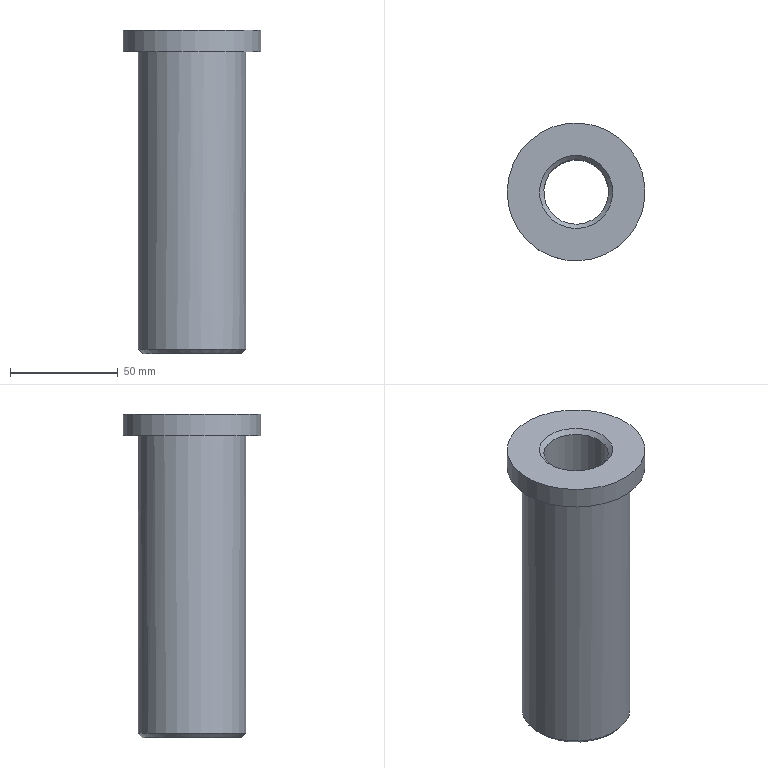Component | NX | PRESSURE_BUSHING | 1 solid | 9 faces | box 64 x 64 x 150 mm | volume 200331 mm3 | plane 3 | cylinder 3 | cone 3 | commonest cylinder face diameters 30 x1 64 x1 50 x1
STEP:
#1=CARTESIAN_POINT('',(0.,0.,0.));
#2=DIRECTION('',(0.,0.,1.));
#3=DIRECTION('',(1.,0.,0.));
#4=AXIS2_PLACEMENT_3D('',#1,#2,#3);
#5=CARTESIAN_POINT('',(-209.297,6.512,90.));
#6=VERTEX_POINT('',#5);
#7=CARTESIAN_POINT('',(-225.,0.,90.));
#8=DIRECTION('',(0.,0.,1.));
#9=DIRECTION('',(0.9237,0.383,0.));
#10=AXIS2_PLACEMENT_3D('',#7,#8,#9);
#11=CIRCLE('',#10,17.);
#12=CARTESIAN_POINT('',(-234.576,23.093,90.));
#13=DIRECTION('',(0.,0.,1.));
#14=DIRECTION('',(0.9237,0.383,0.));
#15=AXIS2_PLACEMENT_3D('',#12,#13,#14);
#16=PLANE('',#15);
#17=CARTESIAN_POINT('',(0.,-25.));
#18=DIRECTION('',(1.,0.));
#19=AXIS2_PLACEMENT_2D('',#17,#18);
#20=CIRCLE('',#19,17.);
#21=(GEOMETRIC_REPRESENTATION_CONTEXT(2)PARAMETRIC_REPRESENTATION_CONTEXT()REPRESENTATION_CONTEXT('',''));
#22=DEFINITIONAL_REPRESENTATION('',(#20),#21);
#23=PCURVE('',#16,#22);
#24=CARTESIAN_POINT('',(-225.,0.,92.));
#25=DIRECTION('',(0.,0.,-1.));
#26=DIRECTION('',(-0.9237,-0.383,0.));
#27=AXIS2_PLACEMENT_3D('',#24,#25,#26);
#28=CONICAL_SURFACE('',#27,15.,0.7854);
#29=CARTESIAN_POINT('',(9.425,2.));
#30=DIRECTION('',(-1.,0.));
#31=VECTOR('',#30,1.);
#32=LINE('',#29,#31);
#33=(GEOMETRIC_REPRESENTATION_CONTEXT(2)PARAMETRIC_REPRESENTATION_CONTEXT()REPRESENTATION_CONTEXT('',''));
#34=DEFINITIONAL_REPRESENTATION('',(#32),#33);
#35=PCURVE('',#28,#34);
#36=SURFACE_CURVE('',#11,(#23,#35),.PCURVE_S1.);
#37=EDGE_CURVE('',#6,#6,#36,.T.);
#38=ORIENTED_EDGE('',*,*,#37,.T.);
#39=EDGE_LOOP('',(#38));
#40=FACE_BOUND('',#39,.T.);
#41=CARTESIAN_POINT('',(-203.754,8.81,90.));
#42=VERTEX_POINT('',#41);
#43=CARTESIAN_POINT('',(-225.,0.,90.));
#44=DIRECTION('',(0.,0.,-1.));
#45=DIRECTION('',(0.9237,0.383,0.));
#46=AXIS2_PLACEMENT_3D('',#43,#44,#45);
#47=CIRCLE('',#46,23.);
#48=CARTESIAN_POINT('',(23.,-25.));
#49=CARTESIAN_POINT('',(23.,-64.837));
#50=CARTESIAN_POINT('',(-11.5,-44.919));
#51=CARTESIAN_POINT('',(-46.,-25.));
#52=CARTESIAN_POINT('',(-11.5,-5.081));
#53=CARTESIAN_POINT('',(23.,14.837));
#54=CARTESIAN_POINT('',(23.,-25.));
#55=(BOUNDED_CURVE()B_SPLINE_CURVE(2,(#48,#49,#50,#51,#52,#53,#54),.UNSPECIFIED.,.T.,.F.)B_SPLINE_CURVE_WITH_KNOTS((1,2,2,2,2,1),(-2.094,0.,2.094,4.189,6.283,8.378),.UNSPECIFIED.)CURVE()GEOMETRIC_REPRESENTATION_ITEM()RATIONAL_B_SPLINE_CURVE((1.,0.5,1.,0.5,1.,0.5,1.))REPRESENTATION_ITEM(''));
#56=(GEOMETRIC_REPRESENTATION_CONTEXT(2)PARAMETRIC_REPRESENTATION_CONTEXT()REPRESENTATION_CONTEXT('',''));
#57=DEFINITIONAL_REPRESENTATION('',(#55),#56);
#58=PCURVE('',#16,#57);
#59=CARTESIAN_POINT('',(-225.,0.,90.));
#60=DIRECTION('',(0.,0.,1.));
#61=DIRECTION('',(0.9237,0.383,0.));
#62=AXIS2_PLACEMENT_3D('',#59,#60,#61);
#63=CONICAL_SURFACE('',#62,23.,0.7854);
#64=CARTESIAN_POINT('',(6.283,-0.));
#65=DIRECTION('',(-1.,0.));
#66=VECTOR('',#65,1.);
#67=LINE('',#64,#66);
#68=(GEOMETRIC_REPRESENTATION_CONTEXT(2)PARAMETRIC_REPRESENTATION_CONTEXT()REPRESENTATION_CONTEXT('',''));
#69=DEFINITIONAL_REPRESENTATION('',(#67),#68);
#70=PCURVE('',#63,#69);
#71=SURFACE_CURVE('',#47,(#58,#70),.PCURVE_S1.);
#72=EDGE_CURVE('',#42,#42,#71,.T.);
#73=ORIENTED_EDGE('',*,*,#72,.T.);
#74=EDGE_LOOP('',(#73));
#75=FACE_BOUND('',#74,.T.);
#76=ADVANCED_FACE('',(#40,#75),#16,.F.);
#77=CARTESIAN_POINT('',(-238.856,-5.746,92.));
#78=VERTEX_POINT('',#77);
#79=CARTESIAN_POINT('',(-211.144,5.746,92.));
#80=VERTEX_POINT('',#79);
#81=CARTESIAN_POINT('',(-225.,0.,92.));
#82=DIRECTION('',(0.,0.,-1.));
#83=DIRECTION('',(0.9237,0.383,0.));
#84=AXIS2_PLACEMENT_3D('',#81,#82,#83);
#85=CIRCLE('',#84,15.);
#86=CARTESIAN_POINT('',(-225.,0.,230.));
#87=DIRECTION('',(0.,0.,-1.));
#88=DIRECTION('',(-0.9237,-0.383,0.));
#89=AXIS2_PLACEMENT_3D('',#86,#87,#88);
#90=CYLINDRICAL_SURFACE('',#89,15.);
#91=CARTESIAN_POINT('',(-3.142,138.));
#92=DIRECTION('',(1.,0.));
#93=VECTOR('',#92,1.);
#94=LINE('',#91,#93);
#95=(GEOMETRIC_REPRESENTATION_CONTEXT(2)PARAMETRIC_REPRESENTATION_CONTEXT()REPRESENTATION_CONTEXT('',''));
#96=DEFINITIONAL_REPRESENTATION('',(#94),#95);
#97=PCURVE('',#90,#96);
#98=CARTESIAN_POINT('',(3.142,0.));
#99=DIRECTION('',(1.,0.));
#100=VECTOR('',#99,1.);
#101=LINE('',#98,#100);
#102=(GEOMETRIC_REPRESENTATION_CONTEXT(2)PARAMETRIC_REPRESENTATION_CONTEXT()REPRESENTATION_CONTEXT('',''));
#103=DEFINITIONAL_REPRESENTATION('',(#101),#102);
#104=PCURVE('',#28,#103);
#105=SURFACE_CURVE('',#85,(#97,#104),.PCURVE_S1.);
#106=EDGE_CURVE('',#78,#80,#105,.T.);
#107=ORIENTED_EDGE('',*,*,#106,.F.);
#108=CARTESIAN_POINT('',(-238.856,-5.746,238.));
#109=VERTEX_POINT('',#108);
#110=CARTESIAN_POINT('',(-238.856,-5.746,238.));
#111=CARTESIAN_POINT('',(-238.856,-5.746,92.));
#112=B_SPLINE_CURVE_WITH_KNOTS('',1,(#110,#111),.UNSPECIFIED.,.F.,.F.,(2,2),(-8.,138.),.PIECEWISE_BEZIER_KNOTS.);
#113=CARTESIAN_POINT('',(0.,0.));
#114=DIRECTION('',(0.,1.));
#115=VECTOR('',#114,1.);
#116=LINE('',#113,#115);
#117=(GEOMETRIC_REPRESENTATION_CONTEXT(2)PARAMETRIC_REPRESENTATION_CONTEXT()REPRESENTATION_CONTEXT('',''));
#118=DEFINITIONAL_REPRESENTATION('',(#116),#117);
#119=PCURVE('',#90,#118);
#120=CARTESIAN_POINT('',(6.283,0.));
#121=DIRECTION('',(0.,1.));
#122=VECTOR('',#121,1.);
#123=LINE('',#120,#122);
#124=(GEOMETRIC_REPRESENTATION_CONTEXT(2)PARAMETRIC_REPRESENTATION_CONTEXT()REPRESENTATION_CONTEXT('',''));
#125=DEFINITIONAL_REPRESENTATION('',(#123),#124);
#126=PCURVE('',#90,#125);
#127=SEAM_CURVE('',#112,(#119,#126),.PCURVE_S1.);
#128=EDGE_CURVE('',#109,#78,#127,.T.);
#129=ORIENTED_EDGE('',*,*,#128,.F.);
#130=CARTESIAN_POINT('',(-225.,0.,238.));
#131=DIRECTION('',(0.,0.,1.));
#132=DIRECTION('',(-0.9237,-0.383,0.));
#133=AXIS2_PLACEMENT_3D('',#130,#131,#132);
#134=CIRCLE('',#133,15.);
#135=CARTESIAN_POINT('',(6.283,-8.));
#136=DIRECTION('',(-1.,0.));
#137=VECTOR('',#136,1.);
#138=LINE('',#135,#137);
#139=(GEOMETRIC_REPRESENTATION_CONTEXT(2)PARAMETRIC_REPRESENTATION_CONTEXT()REPRESENTATION_CONTEXT('',''));
#140=DEFINITIONAL_REPRESENTATION('',(#138),#139);
#141=PCURVE('',#90,#140);
#142=CARTESIAN_POINT('',(-225.,0.,240.));
#143=DIRECTION('',(0.,0.,1.));
#144=DIRECTION('',(0.9237,0.383,0.));
#145=AXIS2_PLACEMENT_3D('',#142,#143,#144);
#146=CONICAL_SURFACE('',#145,17.,0.7854);
#147=CARTESIAN_POINT('',(3.142,-2.));
#148=DIRECTION('',(1.,0.));
#149=VECTOR('',#148,1.);
#150=LINE('',#147,#149);
#151=(GEOMETRIC_REPRESENTATION_CONTEXT(2)PARAMETRIC_REPRESENTATION_CONTEXT()REPRESENTATION_CONTEXT('',''));
#152=DEFINITIONAL_REPRESENTATION('',(#150),#151);
#153=PCURVE('',#146,#152);
#154=SURFACE_CURVE('',#134,(#141,#153),.PCURVE_S1.);
#155=EDGE_CURVE('',#109,#109,#154,.T.);
#156=ORIENTED_EDGE('',*,*,#155,.F.);
#157=ORIENTED_EDGE('',*,*,#128,.T.);
#158=CARTESIAN_POINT('',(-225.,0.,92.));
#159=DIRECTION('',(0.,0.,-1.));
#160=DIRECTION('',(0.9237,0.383,0.));
#161=AXIS2_PLACEMENT_3D('',#158,#159,#160);
#162=CIRCLE('',#161,15.);
#163=CARTESIAN_POINT('',(3.142,138.));
#164=DIRECTION('',(1.,0.));
#165=VECTOR('',#164,1.);
#166=LINE('',#163,#165);
#167=(GEOMETRIC_REPRESENTATION_CONTEXT(2)PARAMETRIC_REPRESENTATION_CONTEXT()REPRESENTATION_CONTEXT('',''));
#168=DEFINITIONAL_REPRESENTATION('',(#166),#167);
#169=PCURVE('',#90,#168);
#170=CARTESIAN_POINT('',(3.142,0.));
#171=DIRECTION('',(1.,0.));
#172=VECTOR('',#171,1.);
#173=LINE('',#170,#172);
#174=(GEOMETRIC_REPRESENTATION_CONTEXT(2)PARAMETRIC_REPRESENTATION_CONTEXT()REPRESENTATION_CONTEXT('',''));
#175=DEFINITIONAL_REPRESENTATION('',(#173),#174);
#176=PCURVE('',#28,#175);
#177=SURFACE_CURVE('',#162,(#169,#176),.PCURVE_S1.);
#178=EDGE_CURVE('',#80,#78,#177,.T.);
#179=ORIENTED_EDGE('',*,*,#178,.F.);
#180=EDGE_LOOP('',(#107,#129,#156,#157,#179));
#181=FACE_BOUND('',#180,.F.);
#182=ADVANCED_FACE('',(#181),#90,.F.);
#183=CARTESIAN_POINT('',(-240.703,-6.512,240.));
#184=VERTEX_POINT('',#183);
#185=CARTESIAN_POINT('',(-225.,0.,240.));
#186=DIRECTION('',(0.,0.,-1.));
#187=DIRECTION('',(-0.9237,-0.383,0.));
#188=AXIS2_PLACEMENT_3D('',#185,#186,#187);
#189=CIRCLE('',#188,17.);
#190=CARTESIAN_POINT('',(-230.746,13.856,240.));
#191=DIRECTION('',(0.,0.,-1.));
#192=DIRECTION('',(-0.9237,-0.383,0.));
#193=AXIS2_PLACEMENT_3D('',#190,#191,#192);
#194=PLANE('',#193);
#195=CARTESIAN_POINT('',(-0.,-15.));
#196=DIRECTION('',(1.,-0.));
#197=AXIS2_PLACEMENT_2D('',#195,#196);
#198=CIRCLE('',#197,17.);
#199=(GEOMETRIC_REPRESENTATION_CONTEXT(2)PARAMETRIC_REPRESENTATION_CONTEXT()REPRESENTATION_CONTEXT('',''));
#200=DEFINITIONAL_REPRESENTATION('',(#198),#199);
#201=PCURVE('',#194,#200);
#202=CARTESIAN_POINT('',(9.425,0.));
#203=DIRECTION('',(-1.,0.));
#204=VECTOR('',#203,1.);
#205=LINE('',#202,#204);
#206=(GEOMETRIC_REPRESENTATION_CONTEXT(2)PARAMETRIC_REPRESENTATION_CONTEXT()REPRESENTATION_CONTEXT('',''));
#207=DEFINITIONAL_REPRESENTATION('',(#205),#206);
#208=PCURVE('',#146,#207);
#209=SURFACE_CURVE('',#189,(#201,#208),.PCURVE_S1.);
#210=EDGE_CURVE('',#184,#184,#209,.T.);
#211=ORIENTED_EDGE('',*,*,#210,.T.);
#212=EDGE_LOOP('',(#211));
#213=FACE_BOUND('',#212,.T.);
#214=CARTESIAN_POINT('',(-254.559,-12.258,240.));
#215=VERTEX_POINT('',#214);
#216=CARTESIAN_POINT('',(-225.,0.,240.));
#217=DIRECTION('',(0.,0.,-1.));
#218=DIRECTION('',(-0.9237,-0.383,0.));
#219=AXIS2_PLACEMENT_3D('',#216,#217,#218);
#220=CIRCLE('',#219,32.);
#221=CARTESIAN_POINT('',(-0.,-15.));
#222=DIRECTION('',(1.,0.));
#223=AXIS2_PLACEMENT_2D('',#221,#222);
#224=CIRCLE('',#223,32.);
#225=(GEOMETRIC_REPRESENTATION_CONTEXT(2)PARAMETRIC_REPRESENTATION_CONTEXT()REPRESENTATION_CONTEXT('',''));
#226=DEFINITIONAL_REPRESENTATION('',(#224),#225);
#227=PCURVE('',#194,#226);
#228=CARTESIAN_POINT('',(-225.,0.,230.));
#229=DIRECTION('',(0.,0.,-1.));
#230=DIRECTION('',(-0.9237,-0.383,0.));
#231=AXIS2_PLACEMENT_3D('',#228,#229,#230);
#232=CYLINDRICAL_SURFACE('',#231,32.);
#233=CARTESIAN_POINT('',(0.,-10.));
#234=DIRECTION('',(1.,0.));
#235=VECTOR('',#234,1.);
#236=LINE('',#233,#235);
#237=(GEOMETRIC_REPRESENTATION_CONTEXT(2)PARAMETRIC_REPRESENTATION_CONTEXT()REPRESENTATION_CONTEXT('',''));
#238=DEFINITIONAL_REPRESENTATION('',(#236),#237);
#239=PCURVE('',#232,#238);
#240=SURFACE_CURVE('',#220,(#227,#239),.PCURVE_S1.);
#241=EDGE_CURVE('',#215,#215,#240,.T.);
#242=ORIENTED_EDGE('',*,*,#241,.F.);
#243=EDGE_LOOP('',(#242));
#244=FACE_BOUND('',#243,.T.);
#245=ADVANCED_FACE('',(#213,#244),#194,.F.);
#246=CARTESIAN_POINT('',(-254.559,-12.258,230.));
#247=VERTEX_POINT('',#246);
#248=CARTESIAN_POINT('',(-225.,0.,230.));
#249=DIRECTION('',(0.,0.,-1.));
#250=DIRECTION('',(-0.9237,-0.383,0.));
#251=AXIS2_PLACEMENT_3D('',#248,#249,#250);
#252=CIRCLE('',#251,32.);
#253=CARTESIAN_POINT('',(0.,0.));
#254=DIRECTION('',(1.,0.));
#255=VECTOR('',#254,1.);
#256=LINE('',#253,#255);
#257=(GEOMETRIC_REPRESENTATION_CONTEXT(2)PARAMETRIC_REPRESENTATION_CONTEXT()REPRESENTATION_CONTEXT('',''));
#258=DEFINITIONAL_REPRESENTATION('',(#256),#257);
#259=PCURVE('',#232,#258);
#260=CARTESIAN_POINT('',(-237.258,29.559,230.));
#261=DIRECTION('',(0.,0.,1.));
#262=DIRECTION('',(0.9237,0.383,0.));
#263=AXIS2_PLACEMENT_3D('',#260,#261,#262);
#264=PLANE('',#263);
#265=CARTESIAN_POINT('',(-32.,-32.));
#266=CARTESIAN_POINT('',(-32.,23.426));
#267=CARTESIAN_POINT('',(16.,-4.287));
#268=CARTESIAN_POINT('',(64.,-32.));
#269=CARTESIAN_POINT('',(16.,-59.713));
#270=CARTESIAN_POINT('',(-32.,-87.426));
#271=CARTESIAN_POINT('',(-32.,-32.));
#272=(BOUNDED_CURVE()B_SPLINE_CURVE(2,(#265,#266,#267,#268,#269,#270,#271),.UNSPECIFIED.,.T.,.F.)B_SPLINE_CURVE_WITH_KNOTS((1,2,2,2,2,1),(-2.094,0.,2.094,4.189,6.283,8.378),.UNSPECIFIED.)CURVE()GEOMETRIC_REPRESENTATION_ITEM()RATIONAL_B_SPLINE_CURVE((1.,0.5,1.,0.5,1.,0.5,1.))REPRESENTATION_ITEM(''));
#273=(GEOMETRIC_REPRESENTATION_CONTEXT(2)PARAMETRIC_REPRESENTATION_CONTEXT()REPRESENTATION_CONTEXT('',''));
#274=DEFINITIONAL_REPRESENTATION('',(#272),#273);
#275=PCURVE('',#264,#274);
#276=SURFACE_CURVE('',#252,(#259,#275),.PCURVE_S1.);
#277=EDGE_CURVE('',#247,#247,#276,.T.);
#278=ORIENTED_EDGE('',*,*,#277,.F.);
#279=CARTESIAN_POINT('',(-254.559,-12.258,240.));
#280=CARTESIAN_POINT('',(-254.559,-12.258,230.));
#281=B_SPLINE_CURVE_WITH_KNOTS('',1,(#279,#280),.UNSPECIFIED.,.F.,.F.,(2,2),(-10.,0.),.PIECEWISE_BEZIER_KNOTS.);
#282=CARTESIAN_POINT('',(0.,0.));
#283=DIRECTION('',(0.,1.));
#284=VECTOR('',#283,1.);
#285=LINE('',#282,#284);
#286=(GEOMETRIC_REPRESENTATION_CONTEXT(2)PARAMETRIC_REPRESENTATION_CONTEXT()REPRESENTATION_CONTEXT('',''));
#287=DEFINITIONAL_REPRESENTATION('',(#285),#286);
#288=PCURVE('',#232,#287);
#289=CARTESIAN_POINT('',(6.283,0.));
#290=DIRECTION('',(0.,1.));
#291=VECTOR('',#290,1.);
#292=LINE('',#289,#291);
#293=(GEOMETRIC_REPRESENTATION_CONTEXT(2)PARAMETRIC_REPRESENTATION_CONTEXT()REPRESENTATION_CONTEXT('',''));
#294=DEFINITIONAL_REPRESENTATION('',(#292),#293);
#295=PCURVE('',#232,#294);
#296=SEAM_CURVE('',#281,(#288,#295),.PCURVE_S1.);
#297=EDGE_CURVE('',#215,#247,#296,.T.);
#298=ORIENTED_EDGE('',*,*,#297,.F.);
#299=ORIENTED_EDGE('',*,*,#241,.T.);
#300=ORIENTED_EDGE('',*,*,#297,.T.);
#301=EDGE_LOOP('',(#278,#298,#299,#300));
#302=FACE_BOUND('',#301,.T.);
#303=ADVANCED_FACE('',(#302),#232,.T.);
#304=CARTESIAN_POINT('',(-248.093,-9.576,230.));
#305=VERTEX_POINT('',#304);
#306=CARTESIAN_POINT('',(-225.,0.,230.));
#307=DIRECTION('',(0.,0.,-1.));
#308=DIRECTION('',(-0.9237,-0.383,0.));
#309=AXIS2_PLACEMENT_3D('',#306,#307,#308);
#310=CIRCLE('',#309,25.);
#311=CARTESIAN_POINT('',(-25.,-32.));
#312=CARTESIAN_POINT('',(-25.,11.301));
#313=CARTESIAN_POINT('',(12.5,-10.349));
#314=CARTESIAN_POINT('',(50.,-32.));
#315=CARTESIAN_POINT('',(12.5,-53.651));
#316=CARTESIAN_POINT('',(-25.,-75.301));
#317=CARTESIAN_POINT('',(-25.,-32.));
#318=(BOUNDED_CURVE()B_SPLINE_CURVE(2,(#311,#312,#313,#314,#315,#316,#317),.UNSPECIFIED.,.T.,.F.)B_SPLINE_CURVE_WITH_KNOTS((1,2,2,2,2,1),(-2.094,0.,2.094,4.189,6.283,8.378),.UNSPECIFIED.)CURVE()GEOMETRIC_REPRESENTATION_ITEM()RATIONAL_B_SPLINE_CURVE((1.,0.5,1.,0.5,1.,0.5,1.))REPRESENTATION_ITEM(''));
#319=(GEOMETRIC_REPRESENTATION_CONTEXT(2)PARAMETRIC_REPRESENTATION_CONTEXT()REPRESENTATION_CONTEXT('',''));
#320=DEFINITIONAL_REPRESENTATION('',(#318),#319);
#321=PCURVE('',#264,#320);
#322=CARTESIAN_POINT('',(-225.,0.,230.));
#323=DIRECTION('',(0.,0.,-1.));
#324=DIRECTION('',(-0.9237,-0.383,0.));
#325=AXIS2_PLACEMENT_3D('',#322,#323,#324);
#326=CYLINDRICAL_SURFACE('',#325,25.);
#327=CARTESIAN_POINT('',(0.,0.));
#328=DIRECTION('',(1.,0.));
#329=VECTOR('',#328,1.);
#330=LINE('',#327,#329);
#331=(GEOMETRIC_REPRESENTATION_CONTEXT(2)PARAMETRIC_REPRESENTATION_CONTEXT()REPRESENTATION_CONTEXT('',''));
#332=DEFINITIONAL_REPRESENTATION('',(#330),#331);
#333=PCURVE('',#326,#332);
#334=SURFACE_CURVE('',#310,(#321,#333),.PCURVE_S1.);
#335=EDGE_CURVE('',#305,#305,#334,.T.);
#336=ORIENTED_EDGE('',*,*,#335,.F.);
#337=EDGE_LOOP('',(#336));
#338=FACE_BOUND('',#337,.T.);
#339=ORIENTED_EDGE('',*,*,#277,.T.);
#340=EDGE_LOOP('',(#339));
#341=FACE_BOUND('',#340,.T.);
#342=ADVANCED_FACE('',(#338,#341),#264,.F.);
#343=CARTESIAN_POINT('',(-201.907,9.576,92.));
#344=VERTEX_POINT('',#343);
#345=CARTESIAN_POINT('',(-248.093,-9.576,92.));
#346=VERTEX_POINT('',#345);
#347=CARTESIAN_POINT('',(-225.,0.,92.));
#348=DIRECTION('',(0.,0.,1.));
#349=DIRECTION('',(0.9237,0.383,0.));
#350=AXIS2_PLACEMENT_3D('',#347,#348,#349);
#351=CIRCLE('',#350,25.);
#352=CARTESIAN_POINT('',(3.142,138.));
#353=DIRECTION('',(-1.,0.));
#354=VECTOR('',#353,1.);
#355=LINE('',#352,#354);
#356=(GEOMETRIC_REPRESENTATION_CONTEXT(2)PARAMETRIC_REPRESENTATION_CONTEXT()REPRESENTATION_CONTEXT('',''));
#357=DEFINITIONAL_REPRESENTATION('',(#355),#356);
#358=PCURVE('',#326,#357);
#359=CARTESIAN_POINT('',(0.,2.));
#360=DIRECTION('',(1.,0.));
#361=VECTOR('',#360,1.);
#362=LINE('',#359,#361);
#363=(GEOMETRIC_REPRESENTATION_CONTEXT(2)PARAMETRIC_REPRESENTATION_CONTEXT()REPRESENTATION_CONTEXT('',''));
#364=DEFINITIONAL_REPRESENTATION('',(#362),#363);
#365=PCURVE('',#63,#364);
#366=SURFACE_CURVE('',#351,(#358,#365),.PCURVE_S1.);
#367=EDGE_CURVE('',#344,#346,#366,.T.);
#368=ORIENTED_EDGE('',*,*,#367,.T.);
#369=CARTESIAN_POINT('',(-248.093,-9.576,230.));
#370=CARTESIAN_POINT('',(-248.093,-9.576,92.));
#371=B_SPLINE_CURVE_WITH_KNOTS('',1,(#369,#370),.UNSPECIFIED.,.F.,.F.,(2,2),(0.,138.),.PIECEWISE_BEZIER_KNOTS.);
#372=CARTESIAN_POINT('',(0.,0.));
#373=DIRECTION('',(0.,1.));
#374=VECTOR('',#373,1.);
#375=LINE('',#372,#374);
#376=(GEOMETRIC_REPRESENTATION_CONTEXT(2)PARAMETRIC_REPRESENTATION_CONTEXT()REPRESENTATION_CONTEXT('',''));
#377=DEFINITIONAL_REPRESENTATION('',(#375),#376);
#378=PCURVE('',#326,#377);
#379=CARTESIAN_POINT('',(6.283,0.));
#380=DIRECTION('',(0.,1.));
#381=VECTOR('',#380,1.);
#382=LINE('',#379,#381);
#383=(GEOMETRIC_REPRESENTATION_CONTEXT(2)PARAMETRIC_REPRESENTATION_CONTEXT()REPRESENTATION_CONTEXT('',''));
#384=DEFINITIONAL_REPRESENTATION('',(#382),#383);
#385=PCURVE('',#326,#384);
#386=SEAM_CURVE('',#371,(#378,#385),.PCURVE_S1.);
#387=EDGE_CURVE('',#305,#346,#386,.T.);
#388=ORIENTED_EDGE('',*,*,#387,.F.);
#389=ORIENTED_EDGE('',*,*,#335,.T.);
#390=ORIENTED_EDGE('',*,*,#387,.T.);
#391=CARTESIAN_POINT('',(-225.,0.,92.));
#392=DIRECTION('',(0.,0.,1.));
#393=DIRECTION('',(0.9237,0.383,0.));
#394=AXIS2_PLACEMENT_3D('',#391,#392,#393);
#395=CIRCLE('',#394,25.);
#396=CARTESIAN_POINT('',(9.425,138.));
#397=DIRECTION('',(-1.,0.));
#398=VECTOR('',#397,1.);
#399=LINE('',#396,#398);
#400=(GEOMETRIC_REPRESENTATION_CONTEXT(2)PARAMETRIC_REPRESENTATION_CONTEXT()REPRESENTATION_CONTEXT('',''));
#401=DEFINITIONAL_REPRESENTATION('',(#399),#400);
#402=PCURVE('',#326,#401);
#403=CARTESIAN_POINT('',(0.,2.));
#404=DIRECTION('',(1.,-0.));
#405=VECTOR('',#404,1.);
#406=LINE('',#403,#405);
#407=(GEOMETRIC_REPRESENTATION_CONTEXT(2)PARAMETRIC_REPRESENTATION_CONTEXT()REPRESENTATION_CONTEXT('',''));
#408=DEFINITIONAL_REPRESENTATION('',(#406),#407);
#409=PCURVE('',#63,#408);
#410=SURFACE_CURVE('',#395,(#402,#409),.PCURVE_S1.);
#411=EDGE_CURVE('',#346,#344,#410,.T.);
#412=ORIENTED_EDGE('',*,*,#411,.T.);
#413=EDGE_LOOP('',(#368,#388,#389,#390,#412));
#414=FACE_BOUND('',#413,.T.);
#415=ADVANCED_FACE('',(#414),#326,.T.);
#416=ORIENTED_EDGE('',*,*,#37,.T.);
#417=CARTESIAN_POINT('',(-211.144,5.746,92.));
#418=CARTESIAN_POINT('',(-209.297,6.512,90.));
#419=B_SPLINE_CURVE_WITH_KNOTS('',1,(#417,#418),.UNSPECIFIED.,.F.,.F.,(2,2),(0.,2.828),.PIECEWISE_BEZIER_KNOTS.);
#420=CARTESIAN_POINT('',(3.142,0.));
#421=DIRECTION('',(0.,1.));
#422=VECTOR('',#421,1.);
#423=LINE('',#420,#422);
#424=(GEOMETRIC_REPRESENTATION_CONTEXT(2)PARAMETRIC_REPRESENTATION_CONTEXT()REPRESENTATION_CONTEXT('',''));
#425=DEFINITIONAL_REPRESENTATION('',(#423),#424);
#426=PCURVE('',#28,#425);
#427=CARTESIAN_POINT('',(9.425,0.));
#428=DIRECTION('',(0.,1.));
#429=VECTOR('',#428,1.);
#430=LINE('',#427,#429);
#431=(GEOMETRIC_REPRESENTATION_CONTEXT(2)PARAMETRIC_REPRESENTATION_CONTEXT()REPRESENTATION_CONTEXT('',''));
#432=DEFINITIONAL_REPRESENTATION('',(#430),#431);
#433=PCURVE('',#28,#432);
#434=SEAM_CURVE('',#419,(#426,#433),.PCURVE_S1.);
#435=EDGE_CURVE('',#80,#6,#434,.T.);
#436=ORIENTED_EDGE('',*,*,#435,.F.);
#437=ORIENTED_EDGE('',*,*,#178,.T.);
#438=ORIENTED_EDGE('',*,*,#106,.T.);
#439=ORIENTED_EDGE('',*,*,#435,.T.);
#440=EDGE_LOOP('',(#416,#436,#437,#438,#439));
#441=FACE_BOUND('',#440,.F.);
#442=ADVANCED_FACE('',(#441),#28,.F.);
#443=ORIENTED_EDGE('',*,*,#367,.F.);
#444=CARTESIAN_POINT('',(-203.754,8.81,90.));
#445=CARTESIAN_POINT('',(-201.907,9.576,92.));
#446=B_SPLINE_CURVE_WITH_KNOTS('',1,(#444,#445),.UNSPECIFIED.,.F.,.F.,(2,2),(-0.,2.828),.PIECEWISE_BEZIER_KNOTS.);
#447=CARTESIAN_POINT('',(0.,0.));
#448=DIRECTION('',(0.,1.));
#449=VECTOR('',#448,1.);
#450=LINE('',#447,#449);
#451=(GEOMETRIC_REPRESENTATION_CONTEXT(2)PARAMETRIC_REPRESENTATION_CONTEXT()REPRESENTATION_CONTEXT('',''));
#452=DEFINITIONAL_REPRESENTATION('',(#450),#451);
#453=PCURVE('',#63,#452);
#454=CARTESIAN_POINT('',(6.283,0.));
#455=DIRECTION('',(0.,1.));
#456=VECTOR('',#455,1.);
#457=LINE('',#454,#456);
#458=(GEOMETRIC_REPRESENTATION_CONTEXT(2)PARAMETRIC_REPRESENTATION_CONTEXT()REPRESENTATION_CONTEXT('',''));
#459=DEFINITIONAL_REPRESENTATION('',(#457),#458);
#460=PCURVE('',#63,#459);
#461=SEAM_CURVE('',#446,(#453,#460),.PCURVE_S1.);
#462=EDGE_CURVE('',#42,#344,#461,.T.);
#463=ORIENTED_EDGE('',*,*,#462,.F.);
#464=ORIENTED_EDGE('',*,*,#72,.F.);
#465=ORIENTED_EDGE('',*,*,#462,.T.);
#466=ORIENTED_EDGE('',*,*,#411,.F.);
#467=EDGE_LOOP('',(#443,#463,#464,#465,#466));
#468=FACE_BOUND('',#467,.T.);
#469=ADVANCED_FACE('',(#468),#63,.T.);
#470=ORIENTED_EDGE('',*,*,#155,.T.);
#471=CARTESIAN_POINT('',(-238.856,-5.746,238.));
#472=CARTESIAN_POINT('',(-240.703,-6.512,240.));
#473=B_SPLINE_CURVE_WITH_KNOTS('',1,(#471,#472),.UNSPECIFIED.,.F.,.F.,(2,2),(-2.828,0.),.PIECEWISE_BEZIER_KNOTS.);
#474=CARTESIAN_POINT('',(9.425,0.));
#475=DIRECTION('',(0.,1.));
#476=VECTOR('',#475,1.);
#477=LINE('',#474,#476);
#478=(GEOMETRIC_REPRESENTATION_CONTEXT(2)PARAMETRIC_REPRESENTATION_CONTEXT()REPRESENTATION_CONTEXT('',''));
#479=DEFINITIONAL_REPRESENTATION('',(#477),#478);
#480=PCURVE('',#146,#479);
#481=CARTESIAN_POINT('',(3.142,0.));
#482=DIRECTION('',(0.,1.));
#483=VECTOR('',#482,1.);
#484=LINE('',#481,#483);
#485=(GEOMETRIC_REPRESENTATION_CONTEXT(2)PARAMETRIC_REPRESENTATION_CONTEXT()REPRESENTATION_CONTEXT('',''));
#486=DEFINITIONAL_REPRESENTATION('',(#484),#485);
#487=PCURVE('',#146,#486);
#488=SEAM_CURVE('',#473,(#480,#487),.PCURVE_S1.);
#489=EDGE_CURVE('',#109,#184,#488,.T.);
#490=ORIENTED_EDGE('',*,*,#489,.T.);
#491=ORIENTED_EDGE('',*,*,#210,.T.);
#492=ORIENTED_EDGE('',*,*,#489,.F.);
#493=EDGE_LOOP('',(#470,#490,#491,#492));
#494=FACE_BOUND('',#493,.F.);
#495=ADVANCED_FACE('',(#494),#146,.F.);
#496=CLOSED_SHELL('',(#76,#182,#245,#303,#342,#415,#442,#469,#495));
#497=MANIFOLD_SOLID_BREP('',#496);
#498=(LENGTH_UNIT()NAMED_UNIT(*)SI_UNIT(.MILLI.,.METRE.));
#499=UNCERTAINTY_MEASURE_WITH_UNIT(LENGTH_MEASURE(0.00001),#498,'','');
#500=(NAMED_UNIT(*)PLANE_ANGLE_UNIT()SI_UNIT($,.RADIAN.));
#501=(NAMED_UNIT(*)SI_UNIT($,.STERADIAN.)SOLID_ANGLE_UNIT());
#502=(GEOMETRIC_REPRESENTATION_CONTEXT(3)GLOBAL_UNCERTAINTY_ASSIGNED_CONTEXT((#499))GLOBAL_UNIT_ASSIGNED_CONTEXT((#498,#500,#501))REPRESENTATION_CONTEXT('',''));
#503=ADVANCED_BREP_SHAPE_REPRESENTATION('',(#4,#497),#502);